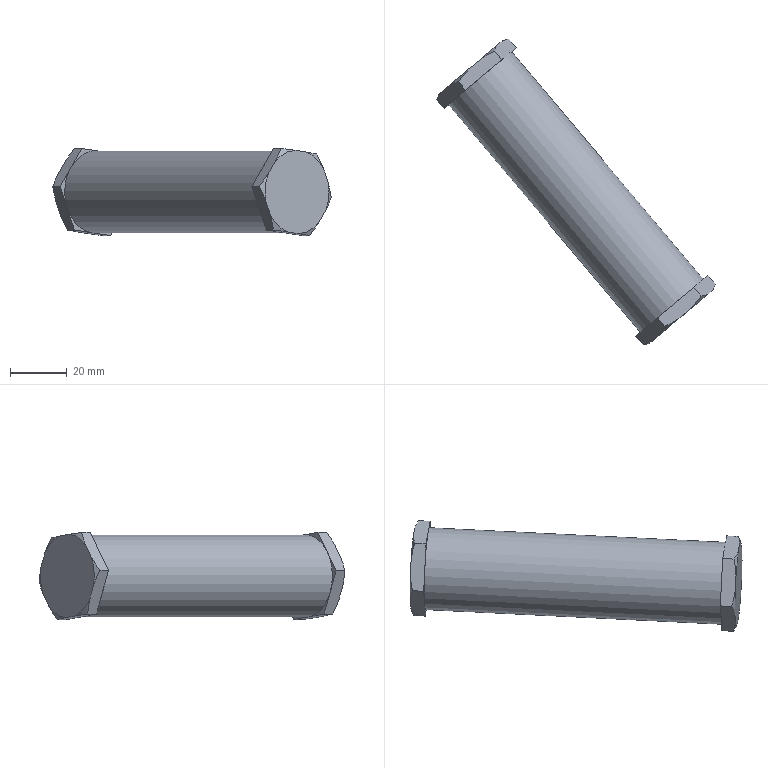Component | NX | PERNO2 | 1 solid | 39 faces | volume 76606 mm3 | plane 26 | cone 12 | cylinder 1 | commonest cylinder face diameters 29 x1